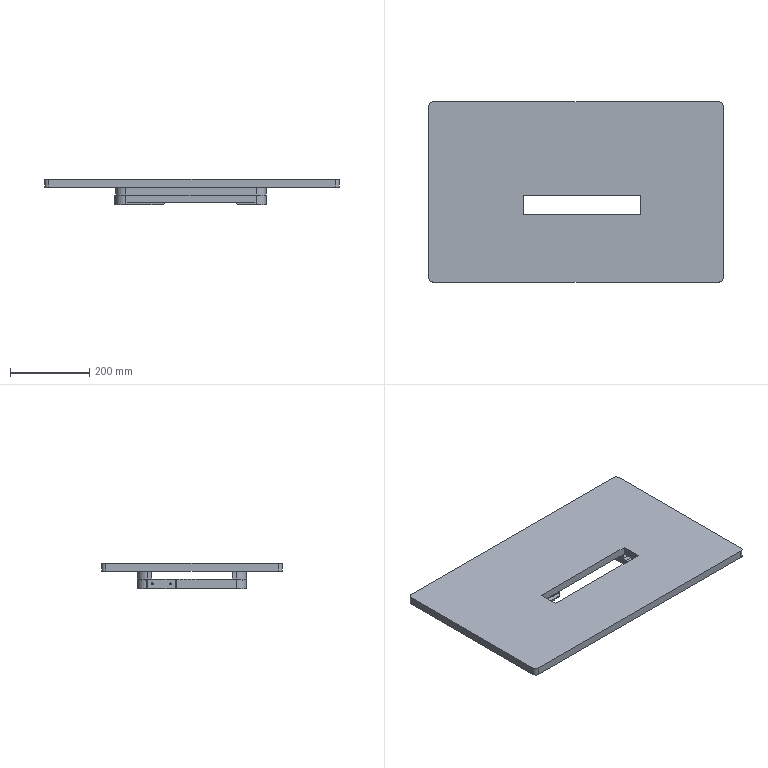Component | SolidWorks | Base-1 | 2 solids | 399 faces | box 740.79 x 454.02 x 64.5 mm | volume 7355354 mm3 | plane 272 | cylinder 92 | torus 15 | spline 10 | cone 8 | sphere 2 | commonest cylinder face diameters 2 x23 20 x12 1 x10 50 x8 8.5 x8 10 x7 6.3 x4 5 x4